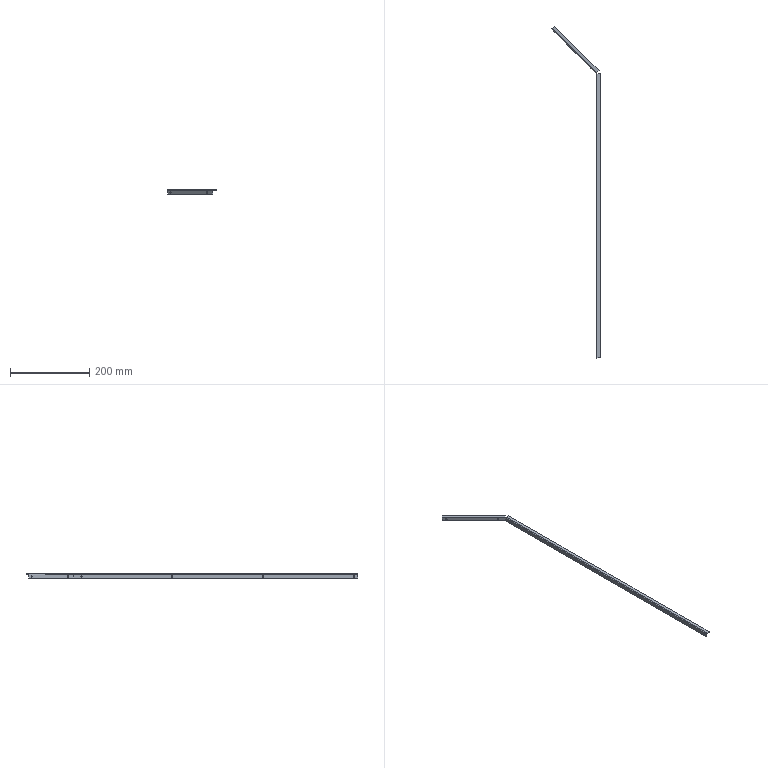Component | SolidWorks | SYM0671-81-300-1_SYM0671-81-302-1 | 1 solid | 44 faces | volume 8532 mm3 | plane 26 | cylinder 18 | commonest cylinder face diameters 3.5 x12 2 x3 3 x3 | material AISI 304